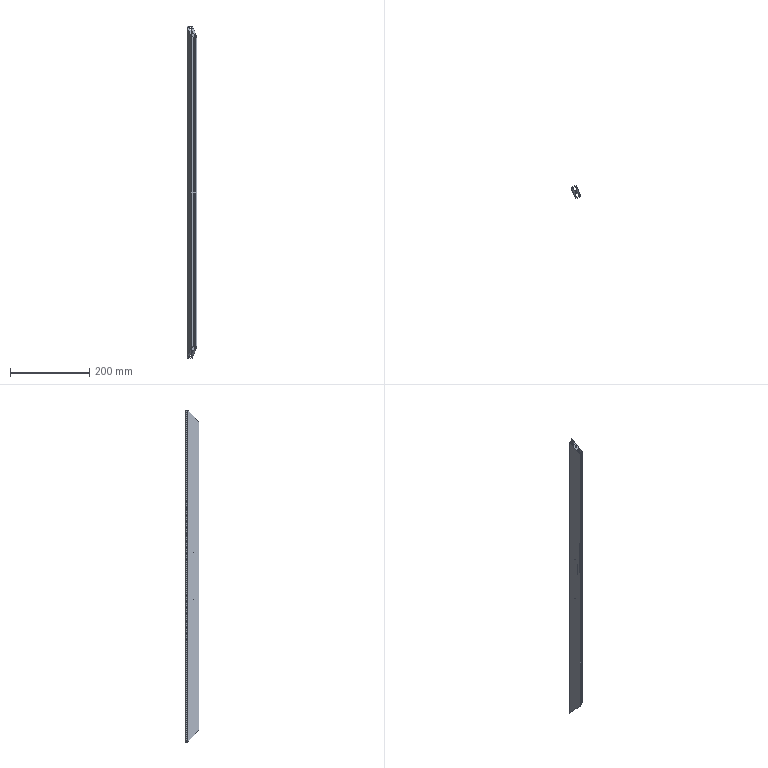Component | SolidWorks | GuardDoor-1_3015-840-1 | 1 solid | 38 faces | box 25.09 x 33.43 x 840 mm | volume 205791 mm3 | plane 32 | cylinder 6 | commonest cylinder face diameters 1 x4 5 x2
build123d program:
from build123d import *

# Parameters (mm, degrees)
SKETCH1_R           = 2.5
BOSS_EXTRUDE1_DEPTH = 840
CUT_EXTRUDE1_DEPTH  = 37
CUT_EXTRUDE2_DEPTH  = 21
SKETCH4_R           = 0.5
CUT_EXTRUDE3_DEPTH  = 0.5


with BuildPart() as part:
    # Sketch1 → Boss-Extrude1 (new body)
    with BuildSketch(Plane.XY):
        Polygon((0, 0), (30, 0), (30, -4.35), (27.5, -4.35), (27.5, -2.35), (22, -2.35), (22, -4.35), (19.5, -4.35), (19.5, -10.65), (22, -10.65), (22, -12.65), (27.5, -12.65), (27.5, -10.65), (30, -10.65), (30, -15), (0, -15), (0, -10.65), (2.5, -10.65), (2.5, -12.65), (8, -12.65), (8, -10.65), (10.5, -10.65), (10.5, -4.35), (8, -4.35), (8, -2.35), (2.5, -2.35), (2.5, -4.35), (0, -4.35), align=None)
        with Locations((15, -7.5)):
            Circle(SKETCH1_R, mode=Mode.SUBTRACT)
    extrude(amount=BOSS_EXTRUDE1_DEPTH)

    # Sketch2 → Cut-Extrude1 (cut)
    with BuildSketch(Plane(origin=(0, 0, 0), x_dir=(1, 0, 0), z_dir=(0, 1, 0))):
        Polygon((30, 0), (30, -30), (0, 0), align=None)
    extrude(amount=-CUT_EXTRUDE1_DEPTH, mode=Mode.SUBTRACT)

    # Sketch3 → Cut-Extrude2 (cut)
    with BuildSketch(Plane(origin=(0, 0, 0), x_dir=(1, 0, 0), z_dir=(0, 1, 0))):
        Polygon((0, -840), (30, -810), (30, -840), align=None)
    extrude(amount=-CUT_EXTRUDE2_DEPTH, mode=Mode.SUBTRACT)

    # Sketch4 → Cut-Extrude3 (cut)
    with BuildSketch(Plane(origin=(0, 0, 0), x_dir=(1, 0, 0), z_dir=(0, 1, 0))):
        with Locations(Location((15, -360, 0), (0, 0, 270))):
            Circle(SKETCH4_R)
        with Locations(Location((15, -480, 0), (0, 0, 270))):
            Circle(SKETCH4_R)
    extrude(amount=-CUT_EXTRUDE3_DEPTH, mode=Mode.SUBTRACT)


solid = part.part

# Placed as in the assembly
solid = solid.moved(Location((861.238, 1157.201, 420), (180, 0, 68.155)))